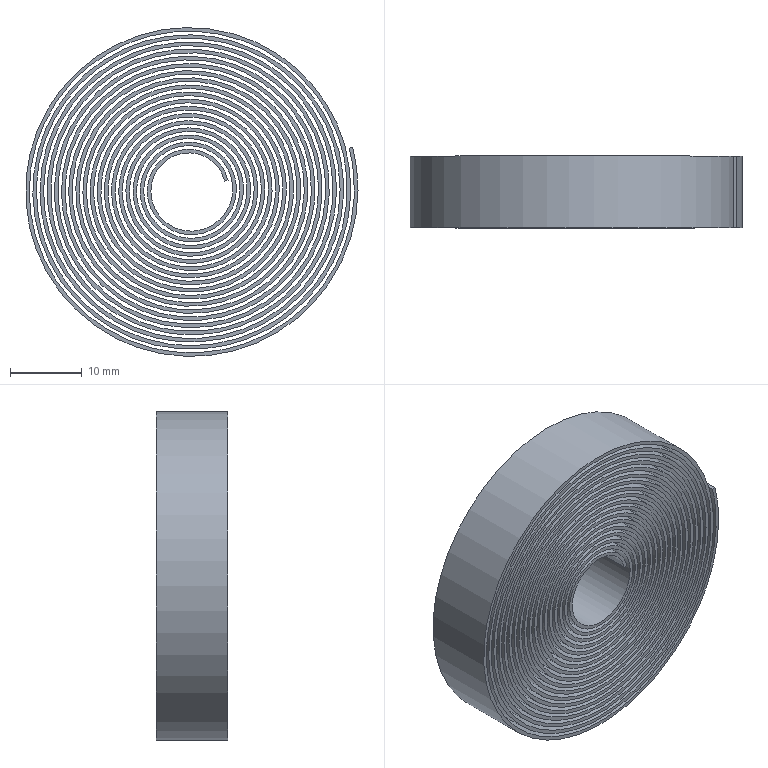Component | SolidWorks | AdhesiveTape-1 | 1 solid | 6 faces | volume 8585 mm3 | plane 4 | spline 2